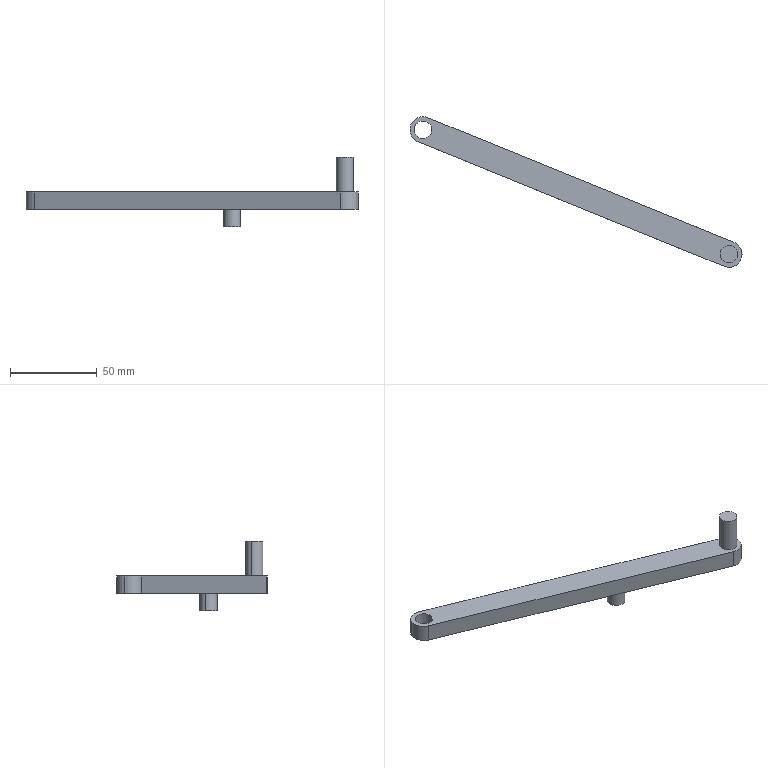Component | SolidWorks | BRocker(Left)-2 | 1 solid | 21 faces | box 190.98 x 86.64 x 40 mm | volume 31068 mm3 | cylinder 13 | plane 8 | commonest cylinder face diameters 10 x6 7 x4 15 x3
build123d program:
from build123d import *

# Parameters (mm, degrees)
BOSS_EXTRUDE1_DEPTH = 10
BOSS_EXTRUDE2_START = 10
SKETCH1_4_R         = 5
BOSS_EXTRUDE2_DEPTH = 20
BOSS_EXTRUDE3_DEPTH = 10
SKETCH2_R           = 5
CUT_EXTRUDE1_DEPTH  = 10
SKETCH3_R           = 3.5
CUT_EXTRUDE2_DEPTH  = 10


with BuildPart() as part:
    # Sketch1_5 → Boss-Extrude1 (new body)
    with BuildSketch(Plane.XY):
        with BuildLine():
            Line((-25.746, 88.007), (-215.746, 88.007))
            ThreePointArc((-215.746, 88.007), (-223.246, 95.507), (-215.746, 103.007))
            Line((-215.746, 103.007), (-25.746, 103.007))
            ThreePointArc((-25.746, 103.007), (-18.246, 95.507), (-25.746, 88.007))
        make_face()
    extrude(amount=BOSS_EXTRUDE1_DEPTH)

    # Sketch1_4 → Boss-Extrude2 (add)
    with BuildSketch(Plane.XY.offset(BOSS_EXTRUDE2_START)):
        with Locations((-25.746, 95.507)):
            Circle(SKETCH1_4_R)
    extrude(amount=BOSS_EXTRUDE2_DEPTH)

    # Sketch1_5 2 → Boss-Extrude3 (add)
    with BuildSketch(Plane.XY):
        with BuildLine():
            ThreePointArc((-100.746, 95.507), (-95.746, 90.507), (-90.746, 95.507))
            Line((-90.746, 95.507), (-100.746, 95.507))
        make_face()
        with BuildLine():
            Line((-100.746, 95.507), (-90.746, 95.507))
            ThreePointArc((-90.746, 95.507), (-95.746, 100.507), (-100.746, 95.507))
        make_face()
        with BuildLine():
            ThreePointArc((-100.746, 95.507), (-95.746, 90.507), (-90.746, 95.507))
            Line((-90.746, 95.507), (-100.746, 95.507))
        make_face()
        with BuildLine():
            Line((-100.746, 95.507), (-90.746, 95.507))
            ThreePointArc((-90.746, 95.507), (-95.746, 100.507), (-100.746, 95.507))
        make_face()
    extrude(amount=-BOSS_EXTRUDE3_DEPTH)

    # Sketch2 → Cut-Extrude1 (cut)
    with BuildSketch(Plane.XY.offset(10)):
        with Locations((-215.746, 95.507)):
            Circle(SKETCH2_R)
    extrude(amount=-CUT_EXTRUDE1_DEPTH, mode=Mode.SUBTRACT)

    # Sketch3 → Cut-Extrude2 (cut)
    with BuildSketch(Plane(origin=(0, 103.007, 0), x_dir=(1, 0, 0), z_dir=(0, 1, 0))):
        with Locations(Location((-195.746, -5, 0), (0, 0, 180))):
            Circle(SKETCH3_R)
        with Locations(Location((-45.746, -5, 0), (0, 0, 180))):
            Circle(SKETCH3_R)
    extrude(amount=-CUT_EXTRUDE2_DEPTH, mode=Mode.SUBTRACT)


solid = part.part

# Placed as in the assembly
solid = solid.moved(Location((-56.396, -122.271, 107.182), (0, 0, -22.15)))
STEP:
#1=CARTESIAN_POINT('',(-7.85,1.431,4.417));
#2=VERTEX_POINT('',#1);
#3=CARTESIAN_POINT('',(-8.105,1.535,4.417));
#4=VERTEX_POINT('',#3);
#5=CARTESIAN_POINT('',(-7.978,1.483,4.417));
#6=DIRECTION('',(0.377,0.9262,-0.));
#7=DIRECTION('',(-0.9262,0.377,0.));
#8=AXIS2_PLACEMENT_3D('',#5,#6,#7);
#9=CIRCLE('',#8,0.1378);
#10=EDGE_CURVE('',#2,#4,#9,.T.);
#11=ORIENTED_EDGE('',*,*,#10,.F.);
#12=CARTESIAN_POINT('',(-7.701,1.796,4.417));
#13=VERTEX_POINT('',#12);
#14=CARTESIAN_POINT('',(-7.85,1.431,4.417));
#15=DIRECTION('',(0.377,0.9262,-0.));
#16=VECTOR('',#15,39.37);
#17=LINE('',#14,#16);
#18=EDGE_CURVE('',#2,#13,#17,.T.);
#19=ORIENTED_EDGE('',*,*,#18,.T.);
#20=CARTESIAN_POINT('',(-7.957,1.9,4.417));
#21=VERTEX_POINT('',#20);
#22=CARTESIAN_POINT('',(-7.829,1.848,4.417));
#23=DIRECTION('',(0.377,0.9262,-0.));
#24=DIRECTION('',(-0.9262,0.377,0.));
#25=AXIS2_PLACEMENT_3D('',#22,#23,#24);
#26=CIRCLE('',#25,0.1378);
#27=EDGE_CURVE('',#13,#21,#26,.T.);
#28=ORIENTED_EDGE('',*,*,#27,.T.);
#29=CARTESIAN_POINT('',(-8.105,1.535,4.417));
#30=DIRECTION('',(0.377,0.9262,-0.));
#31=VECTOR('',#30,39.37);
#32=LINE('',#29,#31);
#33=EDGE_CURVE('',#4,#21,#32,.T.);
#34=ORIENTED_EDGE('',*,*,#33,.F.);
#35=EDGE_LOOP('',(#11,#19,#28,#34));
#36=FACE_OUTER_BOUND('',#35,.T.);
#37=CARTESIAN_POINT('',(-7.978,1.483,4.417));
#38=DIRECTION('',(0.377,0.9262,-0.));
#39=DIRECTION('',(-0.9262,0.377,0.));
#40=AXIS2_PLACEMENT_3D('',#37,#38,#39);
#41=CYLINDRICAL_SURFACE('',#40,0.1378);
#42=ADVANCED_FACE('',(#36),#41,.F.);
#43=CARTESIAN_POINT('',(-2.38,-0.7953,4.417));
#44=VERTEX_POINT('',#43);
#45=CARTESIAN_POINT('',(-2.635,-0.6914,4.417));
#46=VERTEX_POINT('',#45);
#47=CARTESIAN_POINT('',(-2.508,-0.7433,4.417));
#48=DIRECTION('',(0.377,0.9262,-0.));
#49=DIRECTION('',(-0.9262,0.377,0.));
#50=AXIS2_PLACEMENT_3D('',#47,#48,#49);
#51=CIRCLE('',#50,0.1378);
#52=EDGE_CURVE('',#44,#46,#51,.T.);
#53=ORIENTED_EDGE('',*,*,#52,.F.);
#54=CARTESIAN_POINT('',(-2.232,-0.4306,4.417));
#55=VERTEX_POINT('',#54);
#56=CARTESIAN_POINT('',(-2.38,-0.7953,4.417));
#57=DIRECTION('',(0.377,0.9262,-0.));
#58=VECTOR('',#57,39.37);
#59=LINE('',#56,#58);
#60=EDGE_CURVE('',#44,#55,#59,.T.);
#61=ORIENTED_EDGE('',*,*,#60,.T.);
#62=CARTESIAN_POINT('',(-2.487,-0.3267,4.417));
#63=VERTEX_POINT('',#62);
#64=CARTESIAN_POINT('',(-2.359,-0.3787,4.417));
#65=DIRECTION('',(0.377,0.9262,-0.));
#66=DIRECTION('',(-0.9262,0.377,0.));
#67=AXIS2_PLACEMENT_3D('',#64,#65,#66);
#68=CIRCLE('',#67,0.1378);
#69=EDGE_CURVE('',#55,#63,#68,.T.);
#70=ORIENTED_EDGE('',*,*,#69,.T.);
#71=CARTESIAN_POINT('',(-2.635,-0.6914,4.417));
#72=DIRECTION('',(0.377,0.9262,-0.));
#73=VECTOR('',#72,39.37);
#74=LINE('',#71,#73);
#75=EDGE_CURVE('',#46,#63,#74,.T.);
#76=ORIENTED_EDGE('',*,*,#75,.F.);
#77=EDGE_LOOP('',(#53,#61,#70,#76));
#78=FACE_OUTER_BOUND('',#77,.T.);
#79=CARTESIAN_POINT('',(-2.508,-0.7433,4.417));
#80=DIRECTION('',(0.377,0.9262,-0.));
#81=DIRECTION('',(-0.9262,0.377,0.));
#82=AXIS2_PLACEMENT_3D('',#79,#80,#81);
#83=CYLINDRICAL_SURFACE('',#82,0.1378);
#84=ADVANCED_FACE('',(#78),#83,.F.);
#85=CARTESIAN_POINT('',(-8.852,1.946,4.22));
#86=VERTEX_POINT('',#85);
#87=CARTESIAN_POINT('',(-8.487,1.797,4.22));
#88=VERTEX_POINT('',#87);
#89=CARTESIAN_POINT('',(-8.67,1.871,4.22));
#90=DIRECTION('',(-0.,0.,1.));
#91=DIRECTION('',(0.9262,-0.377,0.));
#92=AXIS2_PLACEMENT_3D('',#89,#90,#91);
#93=CIRCLE('',#92,0.1969);
#94=EDGE_CURVE('',#86,#88,#93,.T.);
#95=ORIENTED_EDGE('',*,*,#94,.F.);
#96=CARTESIAN_POINT('',(-8.852,1.946,4.613));
#97=VERTEX_POINT('',#96);
#98=CARTESIAN_POINT('',(-8.852,1.946,4.22));
#99=DIRECTION('',(-0.,0.,1.));
#100=VECTOR('',#99,39.37);
#101=LINE('',#98,#100);
#102=EDGE_CURVE('',#86,#97,#101,.T.);
#103=ORIENTED_EDGE('',*,*,#102,.T.);
#104=CARTESIAN_POINT('',(-8.487,1.797,4.613));
#105=VERTEX_POINT('',#104);
#106=CARTESIAN_POINT('',(-8.67,1.871,4.613));
#107=DIRECTION('',(-0.,0.,1.));
#108=DIRECTION('',(0.9262,-0.377,0.));
#109=AXIS2_PLACEMENT_3D('',#106,#107,#108);
#110=CIRCLE('',#109,0.1969);
#111=EDGE_CURVE('',#97,#105,#110,.T.);
#112=ORIENTED_EDGE('',*,*,#111,.T.);
#113=CARTESIAN_POINT('',(-8.487,1.797,4.22));
#114=DIRECTION('',(-0.,0.,1.));
#115=VECTOR('',#114,39.37);
#116=LINE('',#113,#115);
#117=EDGE_CURVE('',#88,#105,#116,.T.);
#118=ORIENTED_EDGE('',*,*,#117,.F.);
#119=EDGE_LOOP('',(#95,#103,#112,#118));
#120=FACE_OUTER_BOUND('',#119,.T.);
#121=CARTESIAN_POINT('',(-8.67,1.871,4.22));
#122=DIRECTION('',(-0.,0.,1.));
#123=DIRECTION('',(0.9262,-0.377,0.));
#124=AXIS2_PLACEMENT_3D('',#121,#122,#123);
#125=CYLINDRICAL_SURFACE('',#124,0.1969);
#126=ADVANCED_FACE('',(#120),#125,.F.);
#127=CARTESIAN_POINT('',(-4.112,0.01582,3.826));
#128=VERTEX_POINT('',#127);
#129=CARTESIAN_POINT('',(-4.476,0.1643,3.826));
#130=VERTEX_POINT('',#129);
#131=CARTESIAN_POINT('',(-4.294,0.09004,3.826));
#132=DIRECTION('',(-0.,0.,1.));
#133=DIRECTION('',(0.9262,-0.377,0.));
#134=AXIS2_PLACEMENT_3D('',#131,#132,#133);
#135=CIRCLE('',#134,0.1969);
#136=EDGE_CURVE('',#128,#130,#135,.T.);
#137=ORIENTED_EDGE('',*,*,#136,.T.);
#138=CARTESIAN_POINT('',(-4.476,0.1643,4.22));
#139=VERTEX_POINT('',#138);
#140=CARTESIAN_POINT('',(-4.476,0.1643,3.826));
#141=DIRECTION('',(-0.,0.,1.));
#142=VECTOR('',#141,39.37);
#143=LINE('',#140,#142);
#144=EDGE_CURVE('',#130,#139,#143,.T.);
#145=ORIENTED_EDGE('',*,*,#144,.T.);
#146=CARTESIAN_POINT('',(-4.112,0.01582,4.22));
#147=VERTEX_POINT('',#146);
#148=CARTESIAN_POINT('',(-4.294,0.09004,4.22));
#149=DIRECTION('',(-0.,0.,1.));
#150=DIRECTION('',(0.9262,-0.377,0.));
#151=AXIS2_PLACEMENT_3D('',#148,#149,#150);
#152=CIRCLE('',#151,0.1969);
#153=EDGE_CURVE('',#147,#139,#152,.T.);
#154=ORIENTED_EDGE('',*,*,#153,.F.);
#155=CARTESIAN_POINT('',(-4.112,0.01582,3.826));
#156=DIRECTION('',(-0.,0.,1.));
#157=VECTOR('',#156,39.37);
#158=LINE('',#155,#157);
#159=EDGE_CURVE('',#128,#147,#158,.T.);
#160=ORIENTED_EDGE('',*,*,#159,.F.);
#161=EDGE_LOOP('',(#137,#145,#154,#160));
#162=FACE_OUTER_BOUND('',#161,.T.);
#163=CARTESIAN_POINT('',(-4.294,0.09004,3.826));
#164=DIRECTION('',(-0.,0.,1.));
#165=DIRECTION('',(0.9262,-0.377,0.));
#166=AXIS2_PLACEMENT_3D('',#163,#164,#165);
#167=CYLINDRICAL_SURFACE('',#166,0.1969);
#168=ADVANCED_FACE('',(#162),#167,.T.);
#169=CARTESIAN_POINT('',(-1.559,-1.023,5.401));
#170=VERTEX_POINT('',#169);
#171=CARTESIAN_POINT('',(-1.924,-0.8748,5.401));
#172=VERTEX_POINT('',#171);
#173=CARTESIAN_POINT('',(-1.741,-0.949,5.401));
#174=DIRECTION('',(-0.,0.,1.));
#175=DIRECTION('',(0.9262,-0.377,0.));
#176=AXIS2_PLACEMENT_3D('',#173,#174,#175);
#177=CIRCLE('',#176,0.1969);
#178=EDGE_CURVE('',#170,#172,#177,.T.);
#179=ORIENTED_EDGE('',*,*,#178,.F.);
#180=CARTESIAN_POINT('',(-1.559,-1.023,4.613));
#181=VERTEX_POINT('',#180);
#182=CARTESIAN_POINT('',(-1.559,-1.023,5.401));
#183=DIRECTION('',(0.,-0.,-1.));
#184=VECTOR('',#183,39.37);
#185=LINE('',#182,#184);
#186=EDGE_CURVE('',#170,#181,#185,.T.);
#187=ORIENTED_EDGE('',*,*,#186,.T.);
#188=CARTESIAN_POINT('',(-1.924,-0.8748,4.613));
#189=VERTEX_POINT('',#188);
#190=CARTESIAN_POINT('',(-1.741,-0.949,4.613));
#191=DIRECTION('',(-0.,0.,1.));
#192=DIRECTION('',(0.9262,-0.377,0.));
#193=AXIS2_PLACEMENT_3D('',#190,#191,#192);
#194=CIRCLE('',#193,0.1969);
#195=EDGE_CURVE('',#181,#189,#194,.T.);
#196=ORIENTED_EDGE('',*,*,#195,.T.);
#197=CARTESIAN_POINT('',(-1.924,-0.8748,5.401));
#198=DIRECTION('',(0.,-0.,-1.));
#199=VECTOR('',#198,39.37);
#200=LINE('',#197,#199);
#201=EDGE_CURVE('',#172,#189,#200,.T.);
#202=ORIENTED_EDGE('',*,*,#201,.F.);
#203=EDGE_LOOP('',(#179,#187,#196,#202));
#204=FACE_OUTER_BOUND('',#203,.T.);
#205=CARTESIAN_POINT('',(-1.741,-0.949,5.401));
#206=DIRECTION('',(0.,-0.,-1.));
#207=DIRECTION('',(-0.9262,0.377,0.));
#208=AXIS2_PLACEMENT_3D('',#205,#206,#207);
#209=CYLINDRICAL_SURFACE('',#208,0.1969);
#210=ADVANCED_FACE('',(#204),#209,.T.);
#211=CARTESIAN_POINT('',(-8.943,1.983,4.613));
#212=VERTEX_POINT('',#211);
#213=CARTESIAN_POINT('',(-8.781,1.598,4.613));
#214=VERTEX_POINT('',#213);
#215=CARTESIAN_POINT('',(-8.67,1.871,4.613));
#216=DIRECTION('',(-0.,0.,1.));
#217=DIRECTION('',(0.9262,-0.377,0.));
#218=AXIS2_PLACEMENT_3D('',#215,#216,#217);
#219=CIRCLE('',#218,0.2953);
#220=EDGE_CURVE('',#212,#214,#219,.T.);
#221=ORIENTED_EDGE('',*,*,#220,.F.);
#222=CARTESIAN_POINT('',(-8.943,1.983,4.22));
#223=VERTEX_POINT('',#222);
#224=CARTESIAN_POINT('',(-8.943,1.983,4.613));
#225=DIRECTION('',(0.,-0.,-1.));
#226=VECTOR('',#225,39.37);
#227=LINE('',#224,#226);
#228=EDGE_CURVE('',#212,#223,#227,.T.);
#229=ORIENTED_EDGE('',*,*,#228,.T.);
#230=CARTESIAN_POINT('',(-8.781,1.598,4.22));
#231=VERTEX_POINT('',#230);
#232=CARTESIAN_POINT('',(-8.67,1.871,4.22));
#233=DIRECTION('',(-0.,0.,1.));
#234=DIRECTION('',(0.9262,-0.377,0.));
#235=AXIS2_PLACEMENT_3D('',#232,#233,#234);
#236=CIRCLE('',#235,0.2953);
#237=EDGE_CURVE('',#223,#231,#236,.T.);
#238=ORIENTED_EDGE('',*,*,#237,.T.);
#239=CARTESIAN_POINT('',(-8.781,1.598,4.613));
#240=DIRECTION('',(0.,-0.,-1.));
#241=VECTOR('',#240,39.37);
#242=LINE('',#239,#241);
#243=EDGE_CURVE('',#214,#231,#242,.T.);
#244=ORIENTED_EDGE('',*,*,#243,.F.);
#245=EDGE_LOOP('',(#221,#229,#238,#244));
#246=FACE_OUTER_BOUND('',#245,.T.);
#247=CARTESIAN_POINT('',(-8.67,1.871,4.613));
#248=DIRECTION('',(0.,-0.,-1.));
#249=DIRECTION('',(-0.9262,0.377,0.));
#250=AXIS2_PLACEMENT_3D('',#247,#248,#249);
#251=CYLINDRICAL_SURFACE('',#250,0.2953);
#252=ADVANCED_FACE('',(#246),#251,.T.);
#253=CARTESIAN_POINT('',(-8.67,1.871,4.613));
#254=DIRECTION('',(-0.,0.,1.));
#255=DIRECTION('',(0.9262,-0.377,0.));
#256=AXIS2_PLACEMENT_3D('',#253,#254,#255);
#257=CIRCLE('',#256,0.1969);
#258=EDGE_CURVE('',#105,#97,#257,.T.);
#259=ORIENTED_EDGE('',*,*,#258,.F.);
#260=ORIENTED_EDGE('',*,*,#111,.F.);
#261=EDGE_LOOP('',(#259,#260));
#262=FACE_BOUND('',#261,.T.);
#263=CARTESIAN_POINT('',(-1.741,-0.949,4.613));
#264=DIRECTION('',(-0.,0.,1.));
#265=DIRECTION('',(0.9262,-0.377,0.));
#266=AXIS2_PLACEMENT_3D('',#263,#264,#265);
#267=CIRCLE('',#266,0.1969);
#268=EDGE_CURVE('',#189,#181,#267,.T.);
#269=ORIENTED_EDGE('',*,*,#268,.F.);
#270=ORIENTED_EDGE('',*,*,#195,.F.);
#271=EDGE_LOOP('',(#269,#270));
#272=FACE_BOUND('',#271,.T.);
#273=CARTESIAN_POINT('',(-1.63,-0.6755,4.613));
#274=VERTEX_POINT('',#273);
#275=CARTESIAN_POINT('',(-8.558,2.145,4.613));
#276=VERTEX_POINT('',#275);
#277=CARTESIAN_POINT('',(-0.6913,-1.058,4.613));
#278=DIRECTION('',(-0.9262,0.377,-0.));
#279=VECTOR('',#278,39.37);
#280=LINE('',#277,#279);
#281=EDGE_CURVE('',#274,#276,#280,.T.);
#282=ORIENTED_EDGE('',*,*,#281,.T.);
#283=CARTESIAN_POINT('',(-8.67,1.871,4.613));
#284=DIRECTION('',(-0.,0.,1.));
#285=DIRECTION('',(0.9262,-0.377,0.));
#286=AXIS2_PLACEMENT_3D('',#283,#284,#285);
#287=CIRCLE('',#286,0.2953);
#288=EDGE_CURVE('',#276,#212,#287,.T.);
#289=ORIENTED_EDGE('',*,*,#288,.T.);
#290=ORIENTED_EDGE('',*,*,#220,.T.);
#291=CARTESIAN_POINT('',(-1.853,-1.223,4.613));
#292=VERTEX_POINT('',#291);
#293=CARTESIAN_POINT('',(-0.914,-1.605,4.613));
#294=DIRECTION('',(-0.9262,0.377,-0.));
#295=VECTOR('',#294,39.37);
#296=LINE('',#293,#295);
#297=EDGE_CURVE('',#292,#214,#296,.T.);
#298=ORIENTED_EDGE('',*,*,#297,.F.);
#299=CARTESIAN_POINT('',(-1.741,-0.949,4.613));
#300=DIRECTION('',(-0.,0.,1.));
#301=DIRECTION('',(0.9262,-0.377,0.));
#302=AXIS2_PLACEMENT_3D('',#299,#300,#301);
#303=CIRCLE('',#302,0.2953);
#304=EDGE_CURVE('',#292,#274,#303,.T.);
#305=ORIENTED_EDGE('',*,*,#304,.T.);
#306=EDGE_LOOP('',(#282,#289,#290,#298,#305));
#307=FACE_OUTER_BOUND('',#306,.T.);
#308=CARTESIAN_POINT('',(-2.22,-4.814,4.613));
#309=DIRECTION('',(-0.,0.,1.));
#310=DIRECTION('',(0.9262,-0.377,0.));
#311=AXIS2_PLACEMENT_3D('',#308,#309,#310);
#312=PLANE('',#311);
#313=ADVANCED_FACE('',(#262,#272,#307),#312,.T.);
#314=CARTESIAN_POINT('',(-8.67,1.871,4.22));
#315=DIRECTION('',(-0.,0.,1.));
#316=DIRECTION('',(0.9262,-0.377,0.));
#317=AXIS2_PLACEMENT_3D('',#314,#315,#316);
#318=CIRCLE('',#317,0.1969);
#319=EDGE_CURVE('',#88,#86,#318,.T.);
#320=ORIENTED_EDGE('',*,*,#319,.T.);
#321=ORIENTED_EDGE('',*,*,#94,.T.);
#322=EDGE_LOOP('',(#320,#321));
#323=FACE_BOUND('',#322,.T.);
#324=ORIENTED_EDGE('',*,*,#153,.T.);
#325=CARTESIAN_POINT('',(-4.294,0.09004,4.22));
#326=DIRECTION('',(-0.,0.,1.));
#327=DIRECTION('',(0.9262,-0.377,0.));
#328=AXIS2_PLACEMENT_3D('',#325,#326,#327);
#329=CIRCLE('',#328,0.1969);
#330=EDGE_CURVE('',#139,#147,#329,.T.);
#331=ORIENTED_EDGE('',*,*,#330,.T.);
#332=EDGE_LOOP('',(#324,#331));
#333=FACE_BOUND('',#332,.T.);
#334=CARTESIAN_POINT('',(-1.63,-0.6755,4.22));
#335=VERTEX_POINT('',#334);
#336=CARTESIAN_POINT('',(-8.558,2.145,4.22));
#337=VERTEX_POINT('',#336);
#338=CARTESIAN_POINT('',(-0.6913,-1.058,4.22));
#339=DIRECTION('',(-0.9262,0.377,-0.));
#340=VECTOR('',#339,39.37);
#341=LINE('',#338,#340);
#342=EDGE_CURVE('',#335,#337,#341,.T.);
#343=ORIENTED_EDGE('',*,*,#342,.F.);
#344=CARTESIAN_POINT('',(-1.853,-1.223,4.22));
#345=VERTEX_POINT('',#344);
#346=CARTESIAN_POINT('',(-1.741,-0.949,4.22));
#347=DIRECTION('',(-0.,0.,1.));
#348=DIRECTION('',(0.9262,-0.377,0.));
#349=AXIS2_PLACEMENT_3D('',#346,#347,#348);
#350=CIRCLE('',#349,0.2953);
#351=EDGE_CURVE('',#345,#335,#350,.T.);
#352=ORIENTED_EDGE('',*,*,#351,.F.);
#353=CARTESIAN_POINT('',(-0.914,-1.605,4.22));
#354=DIRECTION('',(-0.9262,0.377,-0.));
#355=VECTOR('',#354,39.37);
#356=LINE('',#353,#355);
#357=EDGE_CURVE('',#345,#231,#356,.T.);
#358=ORIENTED_EDGE('',*,*,#357,.T.);
#359=ORIENTED_EDGE('',*,*,#237,.F.);
#360=CARTESIAN_POINT('',(-8.67,1.871,4.22));
#361=DIRECTION('',(-0.,0.,1.));
#362=DIRECTION('',(0.9262,-0.377,0.));
#363=AXIS2_PLACEMENT_3D('',#360,#361,#362);
#364=CIRCLE('',#363,0.2953);
#365=EDGE_CURVE('',#337,#223,#364,.T.);
#366=ORIENTED_EDGE('',*,*,#365,.F.);
#367=EDGE_LOOP('',(#343,#352,#358,#359,#366));
#368=FACE_OUTER_BOUND('',#367,.T.);
#369=CARTESIAN_POINT('',(-2.22,-4.814,4.22));
#370=DIRECTION('',(-0.,0.,1.));
#371=DIRECTION('',(0.9262,-0.377,0.));
#372=AXIS2_PLACEMENT_3D('',#369,#370,#371);
#373=PLANE('',#372);
#374=ADVANCED_FACE('',(#323,#333,#368),#373,.F.);
#375=ORIENTED_EDGE('',*,*,#228,.F.);
#376=ORIENTED_EDGE('',*,*,#288,.F.);
#377=CARTESIAN_POINT('',(-8.558,2.145,4.613));
#378=DIRECTION('',(0.,-0.,-1.));
#379=VECTOR('',#378,39.37);
#380=LINE('',#377,#379);
#381=EDGE_CURVE('',#276,#337,#380,.T.);
#382=ORIENTED_EDGE('',*,*,#381,.T.);
#383=ORIENTED_EDGE('',*,*,#365,.T.);
#384=EDGE_LOOP('',(#375,#376,#382,#383));
#385=FACE_OUTER_BOUND('',#384,.T.);
#386=CARTESIAN_POINT('',(-8.67,1.871,4.613));
#387=DIRECTION('',(0.,-0.,-1.));
#388=DIRECTION('',(-0.9262,0.377,0.));
#389=AXIS2_PLACEMENT_3D('',#386,#387,#388);
#390=CYLINDRICAL_SURFACE('',#389,0.2953);
#391=ADVANCED_FACE('',(#385),#390,.T.);
#392=ORIENTED_EDGE('',*,*,#357,.F.);
#393=CARTESIAN_POINT('',(-1.853,-1.223,4.613));
#394=DIRECTION('',(0.,-0.,-1.));
#395=VECTOR('',#394,39.37);
#396=LINE('',#393,#395);
#397=EDGE_CURVE('',#292,#345,#396,.T.);
#398=ORIENTED_EDGE('',*,*,#397,.F.);
#399=ORIENTED_EDGE('',*,*,#297,.T.);
#400=ORIENTED_EDGE('',*,*,#243,.T.);
#401=EDGE_LOOP('',(#392,#398,#399,#400));
#402=FACE_OUTER_BOUND('',#401,.T.);
#403=CARTESIAN_POINT('',(-0.914,-1.605,4.613));
#404=DIRECTION('',(-0.377,-0.9262,0.));
#405=DIRECTION('',(0.9262,-0.377,0.));
#406=AXIS2_PLACEMENT_3D('',#403,#404,#405);
#407=PLANE('',#406);
#408=ADVANCED_FACE('',(#402),#407,.T.);
#409=ORIENTED_EDGE('',*,*,#351,.T.);
#410=CARTESIAN_POINT('',(-1.63,-0.6755,4.613));
#411=DIRECTION('',(0.,-0.,-1.));
#412=VECTOR('',#411,39.37);
#413=LINE('',#410,#412);
#414=EDGE_CURVE('',#274,#335,#413,.T.);
#415=ORIENTED_EDGE('',*,*,#414,.F.);
#416=ORIENTED_EDGE('',*,*,#304,.F.);
#417=ORIENTED_EDGE('',*,*,#397,.T.);
#418=EDGE_LOOP('',(#409,#415,#416,#417));
#419=FACE_OUTER_BOUND('',#418,.T.);
#420=CARTESIAN_POINT('',(-1.741,-0.949,4.613));
#421=DIRECTION('',(0.,-0.,-1.));
#422=DIRECTION('',(-0.9262,0.377,0.));
#423=AXIS2_PLACEMENT_3D('',#420,#421,#422);
#424=CYLINDRICAL_SURFACE('',#423,0.2953);
#425=ADVANCED_FACE('',(#419),#424,.T.);
#426=CARTESIAN_POINT('',(-7.829,1.848,4.417));
#427=DIRECTION('',(0.377,0.9262,-0.));
#428=DIRECTION('',(-0.9262,0.377,0.));
#429=AXIS2_PLACEMENT_3D('',#426,#427,#428);
#430=CIRCLE('',#429,0.1378);
#431=EDGE_CURVE('',#21,#13,#430,.T.);
#432=ORIENTED_EDGE('',*,*,#431,.F.);
#433=ORIENTED_EDGE('',*,*,#27,.F.);
#434=EDGE_LOOP('',(#432,#433));
#435=FACE_BOUND('',#434,.T.);
#436=CARTESIAN_POINT('',(-2.359,-0.3787,4.417));
#437=DIRECTION('',(0.377,0.9262,-0.));
#438=DIRECTION('',(-0.9262,0.377,0.));
#439=AXIS2_PLACEMENT_3D('',#436,#437,#438);
#440=CIRCLE('',#439,0.1378);
#441=EDGE_CURVE('',#63,#55,#440,.T.);
#442=ORIENTED_EDGE('',*,*,#441,.F.);
#443=ORIENTED_EDGE('',*,*,#69,.F.);
#444=EDGE_LOOP('',(#442,#443));
#445=FACE_BOUND('',#444,.T.);
#446=ORIENTED_EDGE('',*,*,#342,.T.);
#447=ORIENTED_EDGE('',*,*,#381,.F.);
#448=ORIENTED_EDGE('',*,*,#281,.F.);
#449=ORIENTED_EDGE('',*,*,#414,.T.);
#450=EDGE_LOOP('',(#446,#447,#448,#449));
#451=FACE_OUTER_BOUND('',#450,.T.);
#452=CARTESIAN_POINT('',(-0.6913,-1.058,4.613));
#453=DIRECTION('',(-0.377,-0.9262,0.));
#454=DIRECTION('',(0.9262,-0.377,0.));
#455=AXIS2_PLACEMENT_3D('',#452,#453,#454);
#456=PLANE('',#455);
#457=ADVANCED_FACE('',(#435,#445,#451),#456,.F.);
#458=ORIENTED_EDGE('',*,*,#186,.F.);
#459=CARTESIAN_POINT('',(-1.741,-0.949,5.401));
#460=DIRECTION('',(-0.,0.,1.));
#461=DIRECTION('',(0.9262,-0.377,0.));
#462=AXIS2_PLACEMENT_3D('',#459,#460,#461);
#463=CIRCLE('',#462,0.1969);
#464=EDGE_CURVE('',#172,#170,#463,.T.);
#465=ORIENTED_EDGE('',*,*,#464,.F.);
#466=ORIENTED_EDGE('',*,*,#201,.T.);
#467=ORIENTED_EDGE('',*,*,#268,.T.);
#468=EDGE_LOOP('',(#458,#465,#466,#467));
#469=FACE_OUTER_BOUND('',#468,.T.);
#470=CARTESIAN_POINT('',(-1.741,-0.949,5.401));
#471=DIRECTION('',(0.,-0.,-1.));
#472=DIRECTION('',(-0.9262,0.377,0.));
#473=AXIS2_PLACEMENT_3D('',#470,#471,#472);
#474=CYLINDRICAL_SURFACE('',#473,0.1969);
#475=ADVANCED_FACE('',(#469),#474,.T.);
#476=ORIENTED_EDGE('',*,*,#464,.T.);
#477=ORIENTED_EDGE('',*,*,#178,.T.);
#478=EDGE_LOOP('',(#476,#477));
#479=FACE_OUTER_BOUND('',#478,.T.);
#480=CARTESIAN_POINT('',(-1.741,-0.949,5.401));
#481=DIRECTION('',(-0.,0.,1.));
#482=DIRECTION('',(0.9262,-0.377,0.));
#483=AXIS2_PLACEMENT_3D('',#480,#481,#482);
#484=PLANE('',#483);
#485=ADVANCED_FACE('',(#479),#484,.T.);
#486=ORIENTED_EDGE('',*,*,#144,.F.);
#487=CARTESIAN_POINT('',(-4.294,0.09004,3.826));
#488=DIRECTION('',(-0.,0.,1.));
#489=DIRECTION('',(0.9262,-0.377,0.));
#490=AXIS2_PLACEMENT_3D('',#487,#488,#489);
#491=CIRCLE('',#490,0.1969);
#492=EDGE_CURVE('',#130,#128,#491,.T.);
#493=ORIENTED_EDGE('',*,*,#492,.T.);
#494=ORIENTED_EDGE('',*,*,#159,.T.);
#495=ORIENTED_EDGE('',*,*,#330,.F.);
#496=EDGE_LOOP('',(#486,#493,#494,#495));
#497=FACE_OUTER_BOUND('',#496,.T.);
#498=CARTESIAN_POINT('',(-4.294,0.09004,3.826));
#499=DIRECTION('',(-0.,0.,1.));
#500=DIRECTION('',(0.9262,-0.377,0.));
#501=AXIS2_PLACEMENT_3D('',#498,#499,#500);
#502=CYLINDRICAL_SURFACE('',#501,0.1969);
#503=ADVANCED_FACE('',(#497),#502,.T.);
#504=ORIENTED_EDGE('',*,*,#136,.F.);
#505=ORIENTED_EDGE('',*,*,#492,.F.);
#506=EDGE_LOOP('',(#504,#505));
#507=FACE_OUTER_BOUND('',#506,.T.);
#508=CARTESIAN_POINT('',(-2.22,-4.814,3.826));
#509=DIRECTION('',(-0.,0.,1.));
#510=DIRECTION('',(0.9262,-0.377,0.));
#511=AXIS2_PLACEMENT_3D('',#508,#509,#510);
#512=PLANE('',#511);
#513=ADVANCED_FACE('',(#507),#512,.F.);
#514=ORIENTED_EDGE('',*,*,#102,.F.);
#515=ORIENTED_EDGE('',*,*,#319,.F.);
#516=ORIENTED_EDGE('',*,*,#117,.T.);
#517=ORIENTED_EDGE('',*,*,#258,.T.);
#518=EDGE_LOOP('',(#514,#515,#516,#517));
#519=FACE_OUTER_BOUND('',#518,.T.);
#520=CARTESIAN_POINT('',(-8.67,1.871,4.22));
#521=DIRECTION('',(-0.,0.,1.));
#522=DIRECTION('',(0.9262,-0.377,0.));
#523=AXIS2_PLACEMENT_3D('',#520,#521,#522);
#524=CYLINDRICAL_SURFACE('',#523,0.1969);
#525=ADVANCED_FACE('',(#519),#524,.F.);
#526=ORIENTED_EDGE('',*,*,#60,.F.);
#527=CARTESIAN_POINT('',(-2.508,-0.7433,4.417));
#528=DIRECTION('',(0.377,0.9262,-0.));
#529=DIRECTION('',(-0.9262,0.377,0.));
#530=AXIS2_PLACEMENT_3D('',#527,#528,#529);
#531=CIRCLE('',#530,0.1378);
#532=EDGE_CURVE('',#46,#44,#531,.T.);
#533=ORIENTED_EDGE('',*,*,#532,.F.);
#534=ORIENTED_EDGE('',*,*,#75,.T.);
#535=ORIENTED_EDGE('',*,*,#441,.T.);
#536=EDGE_LOOP('',(#526,#533,#534,#535));
#537=FACE_OUTER_BOUND('',#536,.T.);
#538=CARTESIAN_POINT('',(-2.508,-0.7433,4.417));
#539=DIRECTION('',(0.377,0.9262,-0.));
#540=DIRECTION('',(-0.9262,0.377,0.));
#541=AXIS2_PLACEMENT_3D('',#538,#539,#540);
#542=CYLINDRICAL_SURFACE('',#541,0.1378);
#543=ADVANCED_FACE('',(#537),#542,.F.);
#544=ORIENTED_EDGE('',*,*,#532,.T.);
#545=ORIENTED_EDGE('',*,*,#52,.T.);
#546=EDGE_LOOP('',(#544,#545));
#547=FACE_OUTER_BOUND('',#546,.T.);
#548=CARTESIAN_POINT('',(-2.508,-0.7433,4.417));
#549=DIRECTION('',(0.377,0.9262,-0.));
#550=DIRECTION('',(-0.9262,0.377,-0.));
#551=AXIS2_PLACEMENT_3D('',#548,#549,#550);
#552=PLANE('',#551);
#553=ADVANCED_FACE('',(#547),#552,.T.);
#554=ORIENTED_EDGE('',*,*,#18,.F.);
#555=CARTESIAN_POINT('',(-7.978,1.483,4.417));
#556=DIRECTION('',(0.377,0.9262,-0.));
#557=DIRECTION('',(-0.9262,0.377,0.));
#558=AXIS2_PLACEMENT_3D('',#555,#556,#557);
#559=CIRCLE('',#558,0.1378);
#560=EDGE_CURVE('',#4,#2,#559,.T.);
#561=ORIENTED_EDGE('',*,*,#560,.F.);
#562=ORIENTED_EDGE('',*,*,#33,.T.);
#563=ORIENTED_EDGE('',*,*,#431,.T.);
#564=EDGE_LOOP('',(#554,#561,#562,#563));
#565=FACE_OUTER_BOUND('',#564,.T.);
#566=CARTESIAN_POINT('',(-7.978,1.483,4.417));
#567=DIRECTION('',(0.377,0.9262,-0.));
#568=DIRECTION('',(-0.9262,0.377,0.));
#569=AXIS2_PLACEMENT_3D('',#566,#567,#568);
#570=CYLINDRICAL_SURFACE('',#569,0.1378);
#571=ADVANCED_FACE('',(#565),#570,.F.);
#572=ORIENTED_EDGE('',*,*,#560,.T.);
#573=ORIENTED_EDGE('',*,*,#10,.T.);
#574=EDGE_LOOP('',(#572,#573));
#575=FACE_OUTER_BOUND('',#574,.T.);
#576=CARTESIAN_POINT('',(-7.978,1.483,4.417));
#577=DIRECTION('',(0.377,0.9262,-0.));
#578=DIRECTION('',(-0.9262,0.377,-0.));
#579=AXIS2_PLACEMENT_3D('',#576,#577,#578);
#580=PLANE('',#579);
#581=ADVANCED_FACE('',(#575),#580,.T.);
#582=CLOSED_SHELL('',(#42,#84,#126,#168,#210,#252,#313,#374,#391,#408,#425,#457,#475,#485,#503,#513,#525,#543,#553,#571,#581));
#583=MANIFOLD_SOLID_BREP('',#582);
#584=CARTESIAN_POINT('',(0.,0.,0.));
#585=DIRECTION('',(0.,0.,1.));
#586=DIRECTION('',(1.,0.,0.));
#587=AXIS2_PLACEMENT_3D('',#584,#585,#586);
#588=(LENGTH_UNIT()NAMED_UNIT(*)SI_UNIT($,.METRE.));
#589=LENGTH_MEASURE_WITH_UNIT(LENGTH_MEASURE(0.0254),#588);
#590=DIMENSIONAL_EXPONENTS(1.,0.,0.,0.,0.,0.,0.);
#591=(CONVERSION_BASED_UNIT('',#589)LENGTH_UNIT()NAMED_UNIT(#590));
#592=UNCERTAINTY_MEASURE_WITH_UNIT(LENGTH_MEASURE(0.00001),#591,'','');
#593=(NAMED_UNIT(*)PLANE_ANGLE_UNIT()SI_UNIT($,.RADIAN.));
#594=(NAMED_UNIT(*)SI_UNIT($,.STERADIAN.)SOLID_ANGLE_UNIT());
#595=(GEOMETRIC_REPRESENTATION_CONTEXT(3)GLOBAL_UNCERTAINTY_ASSIGNED_CONTEXT((#592))GLOBAL_UNIT_ASSIGNED_CONTEXT((#591,#593,#594))REPRESENTATION_CONTEXT('',''));
#596=ADVANCED_BREP_SHAPE_REPRESENTATION('',(#583,#587),#595);
#597=COLOUR_RGB('',0.7922,0.8196,0.9333);
#598=FILL_AREA_STYLE_COLOUR('',#597);
#599=FILL_AREA_STYLE('',(#598));
#600=SURFACE_STYLE_FILL_AREA(#599);
#601=SURFACE_SIDE_STYLE('',(#600));
#602=SURFACE_STYLE_USAGE(.BOTH.,#601);
#603=PRESENTATION_STYLE_ASSIGNMENT((#602));
#604=STYLED_ITEM('',(#603),#583);
#605=PRESENTATION_LAYER_ASSIGNMENT('','',(#604));
#606=(LENGTH_UNIT()NAMED_UNIT(*)SI_UNIT($,.METRE.));
#607=LENGTH_MEASURE_WITH_UNIT(LENGTH_MEASURE(0.0254),#606);
#608=DIMENSIONAL_EXPONENTS(1.,0.,0.,0.,0.,0.,0.);
#609=(CONVERSION_BASED_UNIT('',#607)LENGTH_UNIT()NAMED_UNIT(#608));
#610=UNCERTAINTY_MEASURE_WITH_UNIT(LENGTH_MEASURE(0.00001),#609,'','');
#611=(NAMED_UNIT(*)PLANE_ANGLE_UNIT()SI_UNIT($,.RADIAN.));
#612=(NAMED_UNIT(*)SI_UNIT($,.STERADIAN.)SOLID_ANGLE_UNIT());
#613=(GEOMETRIC_REPRESENTATION_CONTEXT(3)GLOBAL_UNCERTAINTY_ASSIGNED_CONTEXT((#610))GLOBAL_UNIT_ASSIGNED_CONTEXT((#609,#611,#612))REPRESENTATION_CONTEXT('',''));
#614=MECHANICAL_DESIGN_GEOMETRIC_PRESENTATION_REPRESENTATION('',(#604),#613);